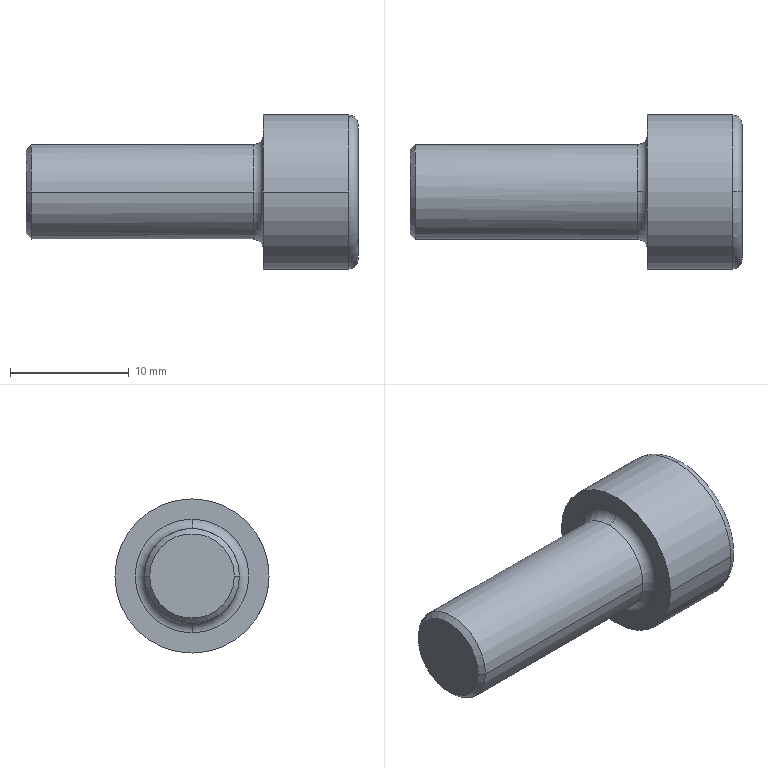Component | NX | M8X20 | 1 solid | 21 faces | volume 1914 mm3 | plane 9 | cylinder 4 | torus 4 | cone 4 | commonest cylinder face diameters 13 x2 8 x2